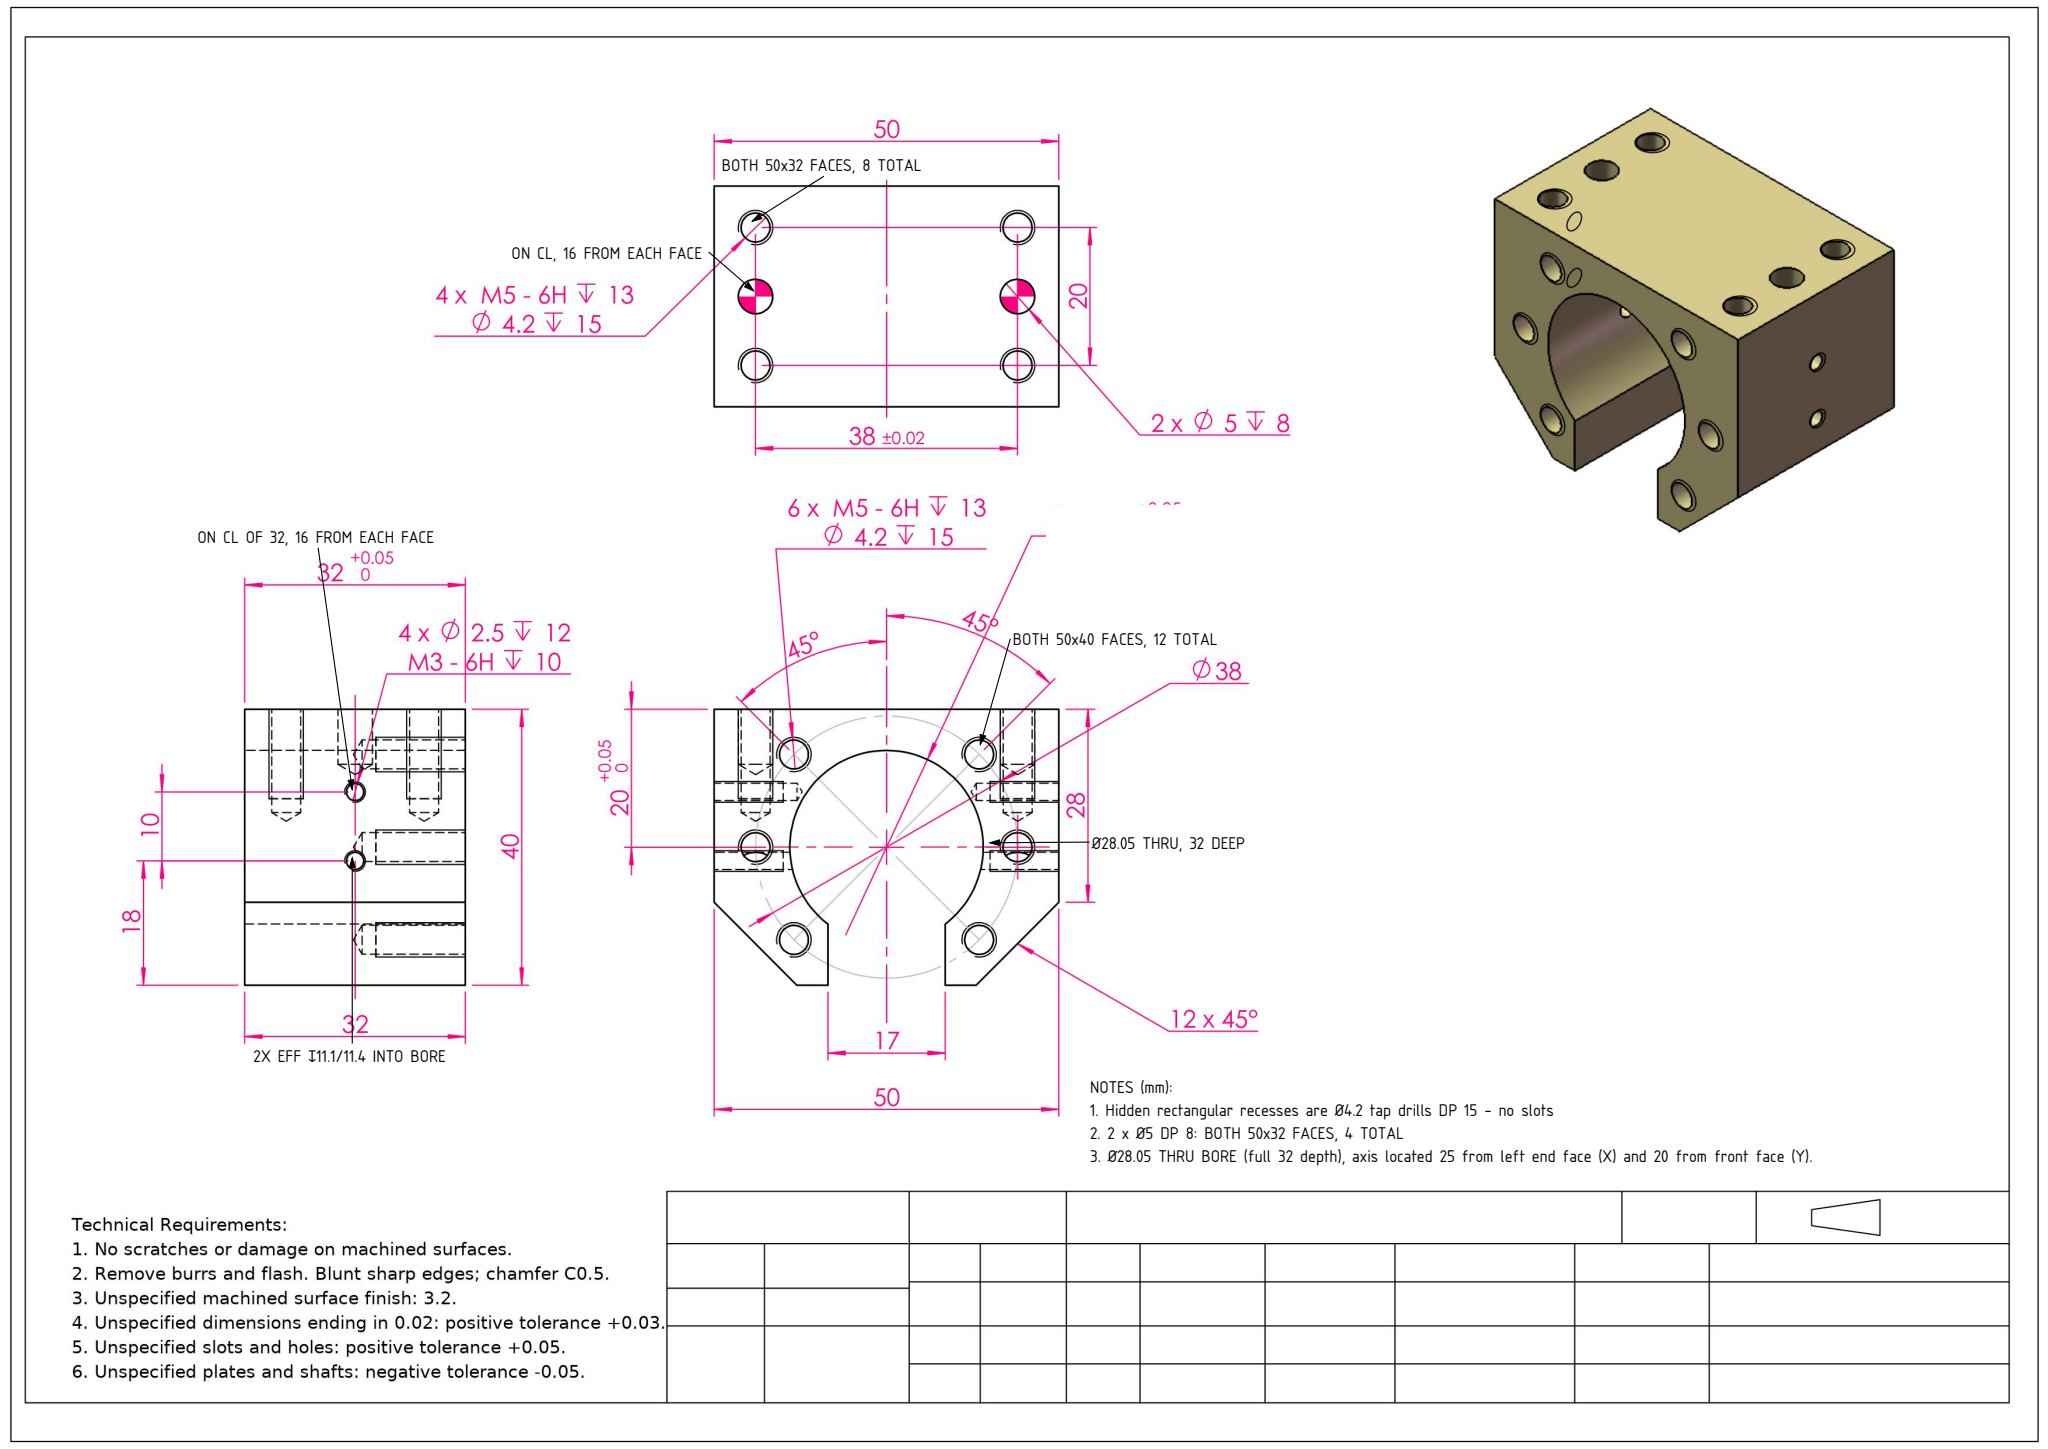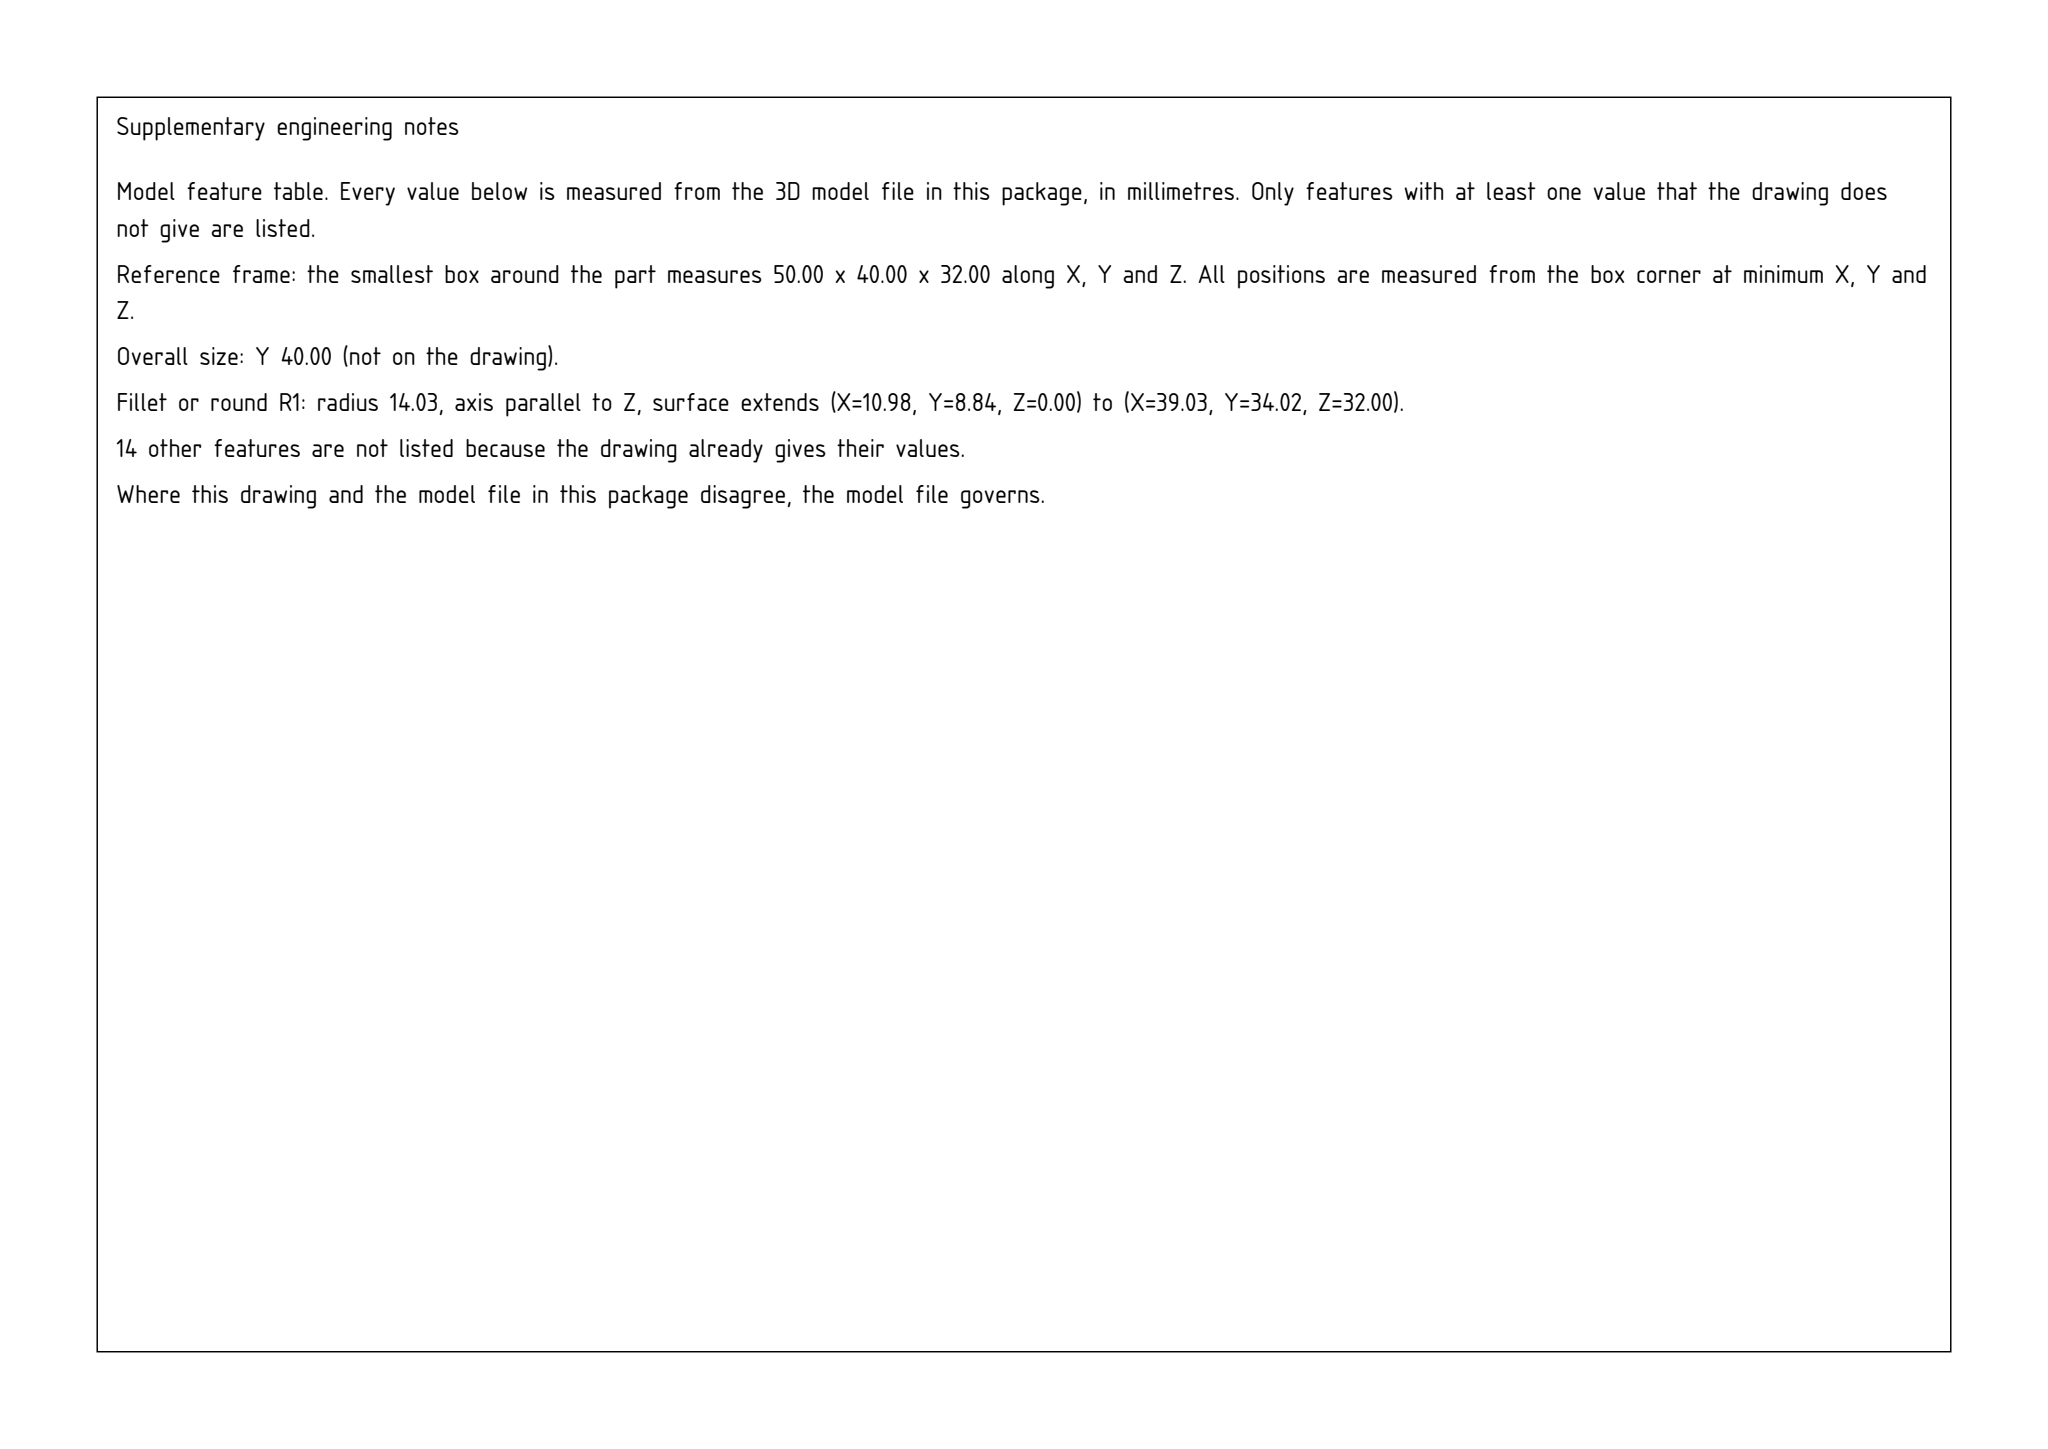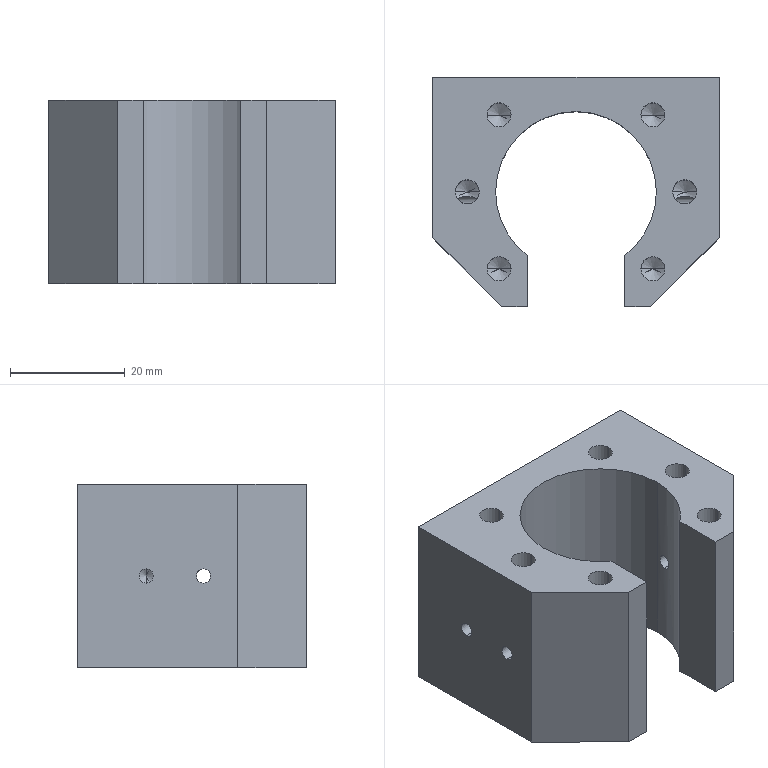Part | SolidWorks | mm | 1 solid | 74 faces | box 50 x 40 x 32 mm | volume 33172 mm3 | cylinder 35 | cone 28 | plane 11 | commonest cylinder face diameters 4.2 x20 2.5 x8 5 x4 28.05 x3
Drawing notes:
4 x Ø2.5 DP 12 / M3-6H DP 10 on CL of 32 width, 16 from each face | from the solid: Ø2.5 cyls, axis x, z=16.0 (32/2), y=18.0 & 28.0; nominal depth 12
2 of the Ø2.5 holes break into Ø28.05 bore (eff. DP 11.12 / 11.36) | from the solid: Ø2.5 cyls lengths 11.12 and 11.36 vs 12.0 for the other pair
Hidden rectangular recesses are Ø4.2 tap drills DP 15 - no slots | from the solid: Ø4.2 cyls len 15 on y axis (6/44, 6/26) and z axis (6/44,20), (11.56/38.44, 6.56/33.44)
2 x Ø5 DP 8 on CL of 32 width, 16 from each face | from the solid: Ø5 cyls, axis y, len 8 at (x6,z16) and (x44,z16)
4 x M5-6H DP 13 / Ø4.2 DP 15: BOTH 50x32 FACES, 8 TOTAL | from the solid: Ø4.2 Y-axis holes at (x,z)=(6,6),(6,26),(44,6),(44,26), count 2 each = 8
2 x Ø5 DP 8: BOTH 50x32 FACES, 4 TOTAL | from the solid: Ø5 Y-axis holes at (x,z)=(6,16),(44,16), count 2 each = 4, L=8
6 x M5-6H DP 13 / Ø4.2 DP 15: BOTH 50x40 FACES, 12 TOTAL | from the solid: Ø4.2 Z-axis holes at (6,20),(44,20),(11.56,6.56),(11.56,33.44),(38.44,6.56),(38.44,33.44), count 2 each = 12
Ø28.05 BORE THRU (32 DEEP), AXIS AT 25 FROM LEFT 50 FACE AND 20 FROM BOTTOM 50x32 FACE | from the solid: cylinders: [28.05,"z",[25.0,20.0],32.0] with bbox_xyz 50x40x32
Ø28.05 THRU BORE (full 32 depth), axis located 25 from left end face (X) and 20 from front face (Y). | from the solid: cylinders[dia,axis,pos_other_axes,length]: [28.05,"z",[25.0,20.0,null],32.0]
build123d program:
from build123d import *

# Parameters (mm, degrees)
SKETCH1_R                     = 14.025
BOSS_EXTRUDE1_DEPTH           = 16
M5_TAPPED_HOLE2_D             = 4.2
M5_TAPPED_HOLE2_DEPTH         = 15
M5_TAPPED_HOLE2_TIP           = 1.262
CUT_EXTRUDE1_DEPTH            = 36.791
CUT_EXTRUDE1_DEPTH_BACK       = 36.791
SKETCH23_W                    = 17
SKETCH23_H                    = 12.022
M5_TAPPED_HOLE1_D             = 4.2
M5_TAPPED_HOLE1_DEPTH         = 15
M5_TAPPED_HOLE1_TIP           = 1.262
M3_TAPPED_HOLE1_AT_2_COUNT    = 2
M3_TAPPED_HOLE1_AT_2_PITCH    = 10
CHAMFER1_SIZE                 = 12
SIZE_MM_DOWEL_PIN_HOLE1_D     = 5
SIZE_MM_DOWEL_PIN_HOLE1_DEPTH = 8
SIZE_MM_DOWEL_PIN_HOLE1_TIP   = 1.502


with BuildPart() as part:
    # Sketch1 → Boss-Extrude1 (new, symmetric)
    with BuildSketch(Plane.XY):
        Polygon((-25, 20), (-25, -20), (0, -20), (25, -20), (25, 20), align=None)
        with Locations(Location((0, 0, 0), (0, 0, 180))):
            Circle(SKETCH1_R, mode=Mode.SUBTRACT)
    extrude(amount=BOSS_EXTRUDE1_DEPTH, both=True)

    # M5 Tapped Hole2
    with Locations(Plane.XY.offset(16)):
        with Locations((-13.435, 13.435), (-19, 0), (-13.435, -13.435), (13.435, 13.435), (19, 0), (13.435, -13.435)):
            Hole(M5_TAPPED_HOLE2_D / 2, depth=M5_TAPPED_HOLE2_DEPTH)
            with Locations((0, 0, -(M5_TAPPED_HOLE2_DEPTH + M5_TAPPED_HOLE2_TIP / 2))):  # 118° drill point
                Cone(0, M5_TAPPED_HOLE2_D / 2, M5_TAPPED_HOLE2_TIP, mode=Mode.SUBTRACT)

    # Sketch23 → Cut-Extrude1 (cut, two sides: drawn at the far end of the back side and taken through both)
    with BuildSketch(Plane.XY.offset(-CUT_EXTRUDE1_DEPTH_BACK)):
        with Locations((0, -17.167)):
            Rectangle(SKETCH23_W, SKETCH23_H)
    extrude(amount=CUT_EXTRUDE1_DEPTH + CUT_EXTRUDE1_DEPTH_BACK, mode=Mode.SUBTRACT)

    # M5 Tapped Hole1
    with Locations(Plane(origin=(0, 20, 0), x_dir=(1, 0, 0), z_dir=(0, 1, 0))):
        with Locations((-19, -10), (-19, 10), (19, -10), (19, 10)):
            Hole(M5_TAPPED_HOLE1_D / 2, depth=M5_TAPPED_HOLE1_DEPTH)
            with Locations((0, 0, -(M5_TAPPED_HOLE1_DEPTH + M5_TAPPED_HOLE1_TIP / 2))):  # 118° drill point
                Cone(0, M5_TAPPED_HOLE1_D / 2, M5_TAPPED_HOLE1_TIP, mode=Mode.SUBTRACT)

    # Sketch34 → M3 Tapped Hole1 (revolve, cut)
    with BuildSketch(Plane(origin=(-25, -2, 0), x_dir=(0, 0, 1), z_dir=(0, 1, 0))):
        Polygon((0, 0), (0, 12.751), (1.25, 12), (1.25, 0), align=None)
    m3_tapped_hole1 = revolve(axis=Axis((-31.35, -2, 0), (1, 0, 0)), mode=Mode.SUBTRACT)

    # M3 Tapped Hole1 at 2: M3 Tapped Hole1 ×2
    with Locations(*[(0, i * M3_TAPPED_HOLE1_AT_2_PITCH, 0) for i in range(1, M3_TAPPED_HOLE1_AT_2_COUNT)]):
        add(m3_tapped_hole1, mode=Mode.SUBTRACT)

    # Mirror1: M3 Tapped Hole1 across plane
    add(m3_tapped_hole1.mirror(Plane(origin=(0, 0, 0), x_dir=(0, 0, 1), z_dir=(1, 0, 0))), mode=Mode.SUBTRACT)

    # Mirror1 copy 1 sketch → Mirror1 copy 1 (revolve, cut)
    with BuildSketch(Plane(origin=(25, 8, 0), x_dir=(0, 0, 1), z_dir=(0, 1, 0))):
        Polygon((0, 0), (0, -12.751), (1.25, -12), (1.25, 0), align=None)
    revolve(axis=Axis((31.35, 8, 0), (1, 0, 0)), mode=Mode.SUBTRACT)

    # Chamfer1
    chamfer1_edges = [part.edges().sort_by_distance(p)[0] for p in [
        (25, -20, 0),
        (-25, -20, 0),
    ]]
    chamfer(chamfer1_edges, length=CHAMFER1_SIZE)

    # Size mm Dowel Pin Hole1
    with Locations(Plane(origin=(0, 20, 0), x_dir=(1, 0, 0), z_dir=(0, 1, 0))):
        with Locations((19, 0), (-19, 0)):
            Hole(SIZE_MM_DOWEL_PIN_HOLE1_D / 2, depth=SIZE_MM_DOWEL_PIN_HOLE1_DEPTH)
            with Locations((0, 0, -(SIZE_MM_DOWEL_PIN_HOLE1_DEPTH + SIZE_MM_DOWEL_PIN_HOLE1_TIP / 2))):  # 118° drill point
                Cone(0, SIZE_MM_DOWEL_PIN_HOLE1_D / 2, SIZE_MM_DOWEL_PIN_HOLE1_TIP, mode=Mode.SUBTRACT)


solid = part.part